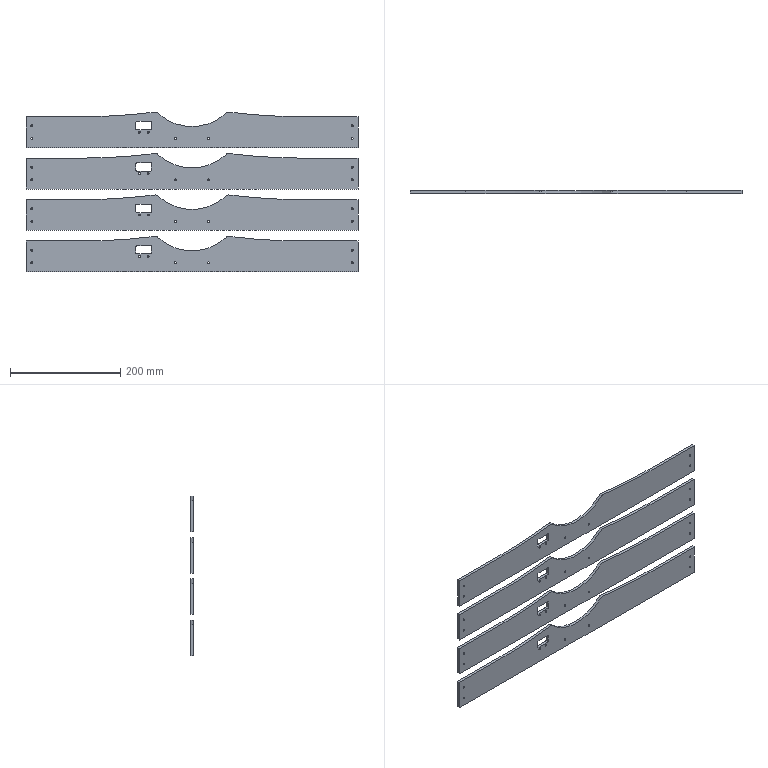CAM job | Mastercam | mm | 4 operations | part box 601 x 5 x 289.35
1. Contour (Ramp) | 3 - 3 平铣刀
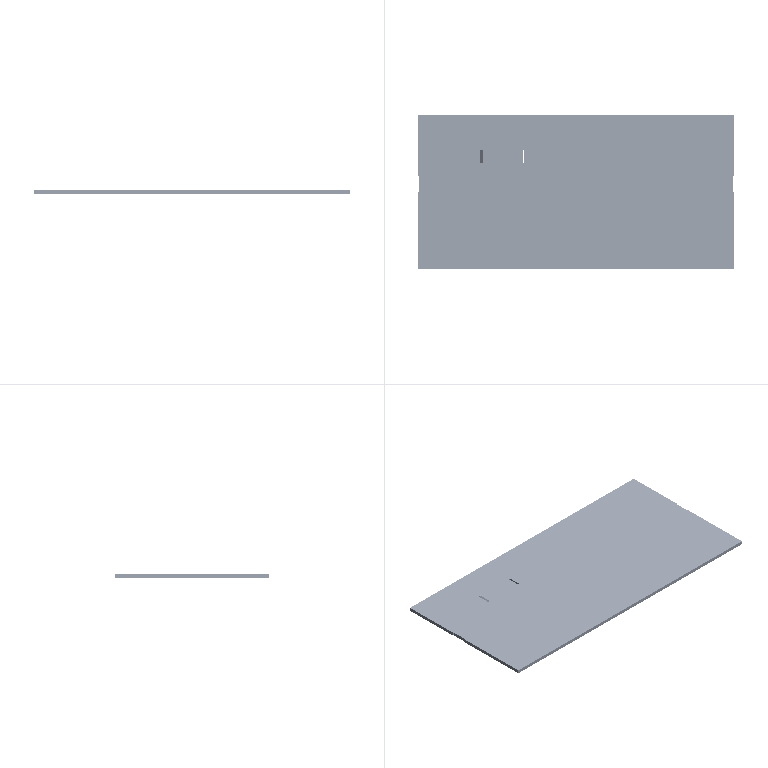2. Contour (2D) | 3 - 3 平铣刀
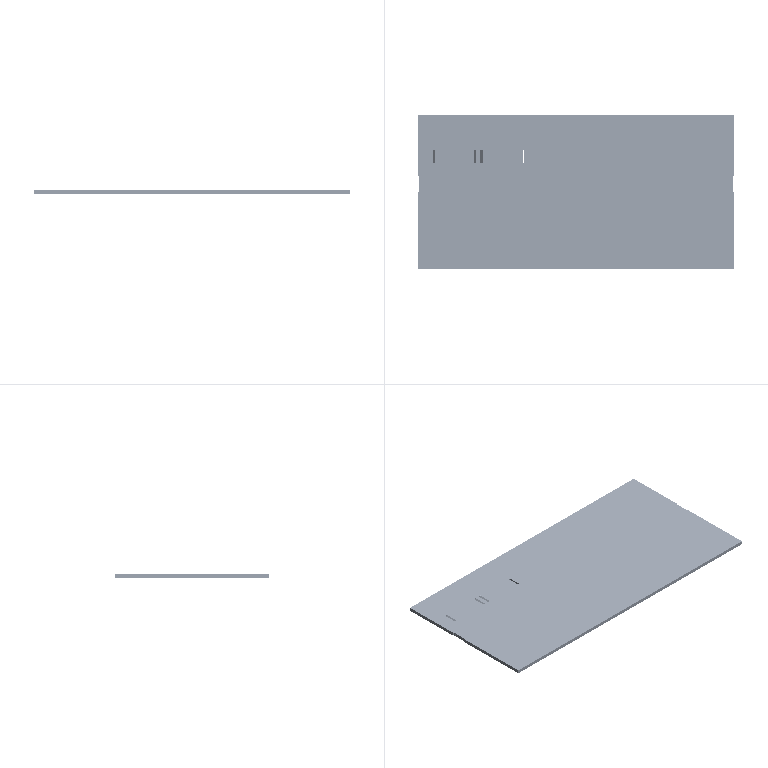3. Drill/Counterbore | 7 - 4 倒角刀
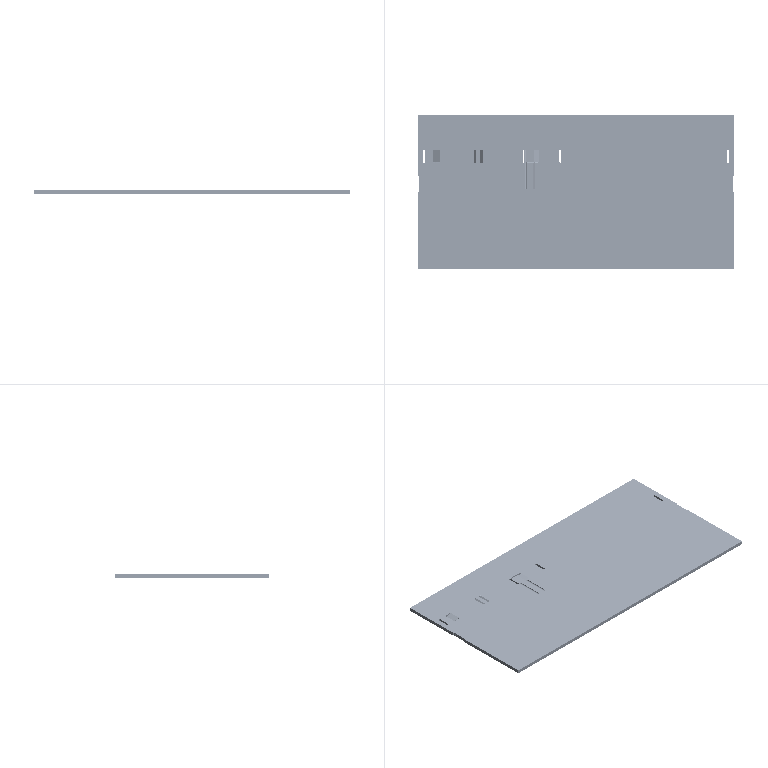4. Contour (2D chamfer) | 7 - 4 倒角刀